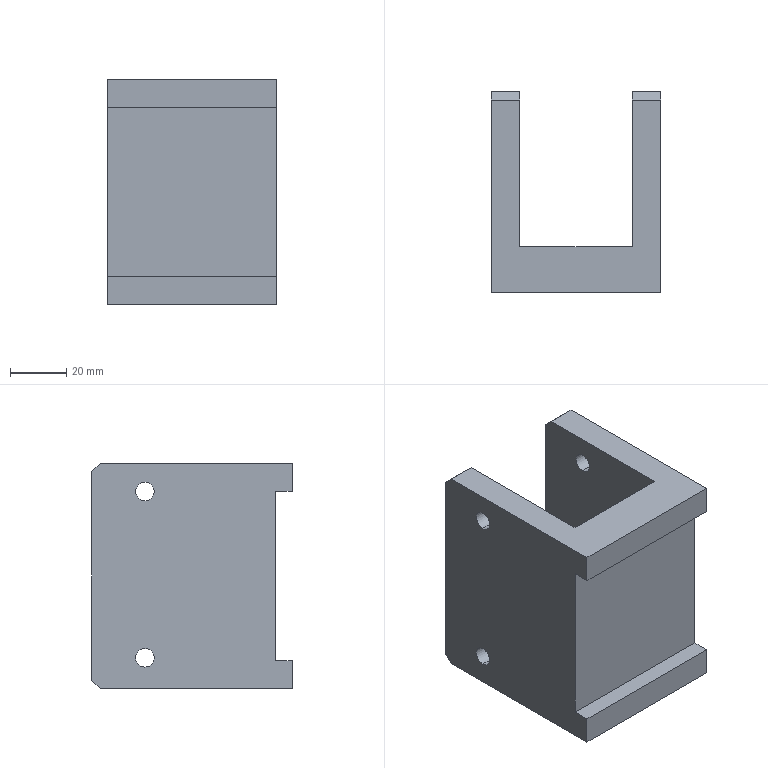Component | SolidWorks | CHEN123-AA-07-1 | 1 solid | 26 faces | box 60 x 71 x 80 mm | volume 141652 mm3 | plane 18 | cylinder 8 | commonest cylinder face diameters 6.6 x8
build123d program:
from build123d import *

# Parameters (mm, degrees)
BOSS_EXTRUDE1_DEPTH        = 80
SKETCH2_W                  = 60
SKETCH2_H                  = 6
CUT_EXTRUDE1_DEPTH         = 123.642
CHAMFER1_SIZE              = 3
F_6_6_6_6_DIAMETER_HOLE1_D = 6.6


with BuildPart() as part:
    # Sketch1 → Boss-Extrude1 (new body)
    with BuildSketch(Plane.XY):
        Polygon((-30, 0), (30, 0), (30, 71), (20, 71), (20, 16), (-20, 16), (-20, 71), (-30, 71), align=None)
    extrude(amount=BOSS_EXTRUDE1_DEPTH)

    # Sketch2 → Cut-Extrude1 (cut, through all)
    with BuildSketch(Plane.ZY.offset(30)):
        with Locations((40, 3)):
            Rectangle(SKETCH2_W, SKETCH2_H)
    extrude(amount=-CUT_EXTRUDE1_DEPTH, mode=Mode.SUBTRACT)

    # Chamfer1
    chamfer1_edges = [part.edges().sort_by_distance(p)[0] for p in [
        (25, 71, 80),
        (-25, 71, 80),
        (-25, 71, 0),
        (25, 71, 0),
    ]]
    chamfer(chamfer1_edges, length=CHAMFER1_SIZE)

    # 6.6 _6.6_ Diameter Hole1 (through all)
    with Locations(Plane(origin=(30, 0, 0), x_dir=(0, 0, -1), z_dir=(1, 0, 0))):
        with Locations((-69.874, 52.155), (-11.032, 52.155)):
            Hole(F_6_6_6_6_DIAMETER_HOLE1_D / 2)


solid = part.part

# Placed as in the assembly
solid = solid.moved(Location((-0.0005, -51.999, -137), (0, 0, 0)))
STEP:
#1=COLOUR_RGB('',0.7922,0.8196,0.9333);
#2=FILL_AREA_STYLE_COLOUR('',#1);
#3=FILL_AREA_STYLE('',(#2));
#4=SURFACE_STYLE_FILL_AREA(#3);
#5=SURFACE_SIDE_STYLE('',(#4));
#6=SURFACE_STYLE_USAGE(.BOTH.,#5);
#7=PRESENTATION_STYLE_ASSIGNMENT((#6));
#8=CARTESIAN_POINT('',(-1.181,0.006131,-2.513));
#9=VERTEX_POINT('',#8);
#10=CARTESIAN_POINT('',(-1.181,0.006131,-2.773));
#11=VERTEX_POINT('',#10);
#12=CARTESIAN_POINT('',(-1.181,0.006131,-2.643));
#13=DIRECTION('',(1.,0.,0.));
#14=DIRECTION('',(0.,0.,-1.));
#15=AXIS2_PLACEMENT_3D('',#12,#13,#14);
#16=CIRCLE('',#15,0.1299);
#17=EDGE_CURVE('',#9,#11,#16,.T.);
#18=ORIENTED_EDGE('',*,*,#17,.F.);
#19=CARTESIAN_POINT('',(-0.7874,0.006131,-2.513));
#20=VERTEX_POINT('',#19);
#21=CARTESIAN_POINT('',(1.181,0.006131,-2.513));
#22=DIRECTION('',(1.,0.,0.));
#23=VECTOR('',#22,39.37);
#24=LINE('',#21,#23);
#25=EDGE_CURVE('',#9,#20,#24,.T.);
#26=ORIENTED_EDGE('',*,*,#25,.T.);
#27=CARTESIAN_POINT('',(-0.7874,0.006131,-2.773));
#28=VERTEX_POINT('',#27);
#29=CARTESIAN_POINT('',(-0.7874,0.006131,-2.643));
#30=DIRECTION('',(-1.,0.,0.));
#31=DIRECTION('',(0.,0.,1.));
#32=AXIS2_PLACEMENT_3D('',#29,#30,#31);
#33=CIRCLE('',#32,0.1299);
#34=EDGE_CURVE('',#28,#20,#33,.T.);
#35=ORIENTED_EDGE('',*,*,#34,.F.);
#36=CARTESIAN_POINT('',(1.181,0.006131,-2.773));
#37=DIRECTION('',(1.,0.,0.));
#38=VECTOR('',#37,39.37);
#39=LINE('',#36,#38);
#40=EDGE_CURVE('',#11,#28,#39,.T.);
#41=ORIENTED_EDGE('',*,*,#40,.F.);
#42=EDGE_LOOP('',(#18,#26,#35,#41));
#43=FACE_OUTER_BOUND('',#42,.T.);
#44=CARTESIAN_POINT('',(1.181,0.006131,-2.643));
#45=DIRECTION('',(1.,0.,0.));
#46=DIRECTION('',(0.,0.,-1.));
#47=AXIS2_PLACEMENT_3D('',#44,#45,#46);
#48=CYLINDRICAL_SURFACE('',#47,0.1299);
#49=ADVANCED_FACE('',(#43),#48,.F.);
#50=CARTESIAN_POINT('',(0.7874,0.006131,-2.513));
#51=VERTEX_POINT('',#50);
#52=CARTESIAN_POINT('',(0.7874,0.006131,-2.773));
#53=VERTEX_POINT('',#52);
#54=CARTESIAN_POINT('',(0.7874,0.006131,-2.643));
#55=DIRECTION('',(1.,0.,0.));
#56=DIRECTION('',(0.,0.,-1.));
#57=AXIS2_PLACEMENT_3D('',#54,#55,#56);
#58=CIRCLE('',#57,0.1299);
#59=EDGE_CURVE('',#51,#53,#58,.T.);
#60=ORIENTED_EDGE('',*,*,#59,.F.);
#61=CARTESIAN_POINT('',(1.181,0.006131,-2.513));
#62=VERTEX_POINT('',#61);
#63=CARTESIAN_POINT('',(1.181,0.006131,-2.513));
#64=DIRECTION('',(1.,0.,0.));
#65=VECTOR('',#64,39.37);
#66=LINE('',#63,#65);
#67=EDGE_CURVE('',#51,#62,#66,.T.);
#68=ORIENTED_EDGE('',*,*,#67,.T.);
#69=CARTESIAN_POINT('',(1.181,0.006131,-2.773));
#70=VERTEX_POINT('',#69);
#71=CARTESIAN_POINT('',(1.181,0.006131,-2.643));
#72=DIRECTION('',(1.,0.,0.));
#73=DIRECTION('',(0.,0.,-1.));
#74=AXIS2_PLACEMENT_3D('',#71,#72,#73);
#75=CIRCLE('',#74,0.1299);
#76=EDGE_CURVE('',#62,#70,#75,.T.);
#77=ORIENTED_EDGE('',*,*,#76,.T.);
#78=CARTESIAN_POINT('',(1.181,0.006131,-2.773));
#79=DIRECTION('',(1.,0.,0.));
#80=VECTOR('',#79,39.37);
#81=LINE('',#78,#80);
#82=EDGE_CURVE('',#53,#70,#81,.T.);
#83=ORIENTED_EDGE('',*,*,#82,.F.);
#84=EDGE_LOOP('',(#60,#68,#77,#83));
#85=FACE_OUTER_BOUND('',#84,.T.);
#86=CARTESIAN_POINT('',(1.181,0.006131,-2.643));
#87=DIRECTION('',(1.,0.,0.));
#88=DIRECTION('',(0.,0.,-1.));
#89=AXIS2_PLACEMENT_3D('',#86,#87,#88);
#90=CYLINDRICAL_SURFACE('',#89,0.1299);
#91=ADVANCED_FACE('',(#85),#90,.F.);
#92=CARTESIAN_POINT('',(0.7874,0.006131,-4.829));
#93=VERTEX_POINT('',#92);
#94=CARTESIAN_POINT('',(0.7874,0.006131,-5.089));
#95=VERTEX_POINT('',#94);
#96=CARTESIAN_POINT('',(0.7874,0.006131,-4.959));
#97=DIRECTION('',(1.,0.,0.));
#98=DIRECTION('',(0.,0.,-1.));
#99=AXIS2_PLACEMENT_3D('',#96,#97,#98);
#100=CIRCLE('',#99,0.1299);
#101=EDGE_CURVE('',#93,#95,#100,.T.);
#102=ORIENTED_EDGE('',*,*,#101,.F.);
#103=CARTESIAN_POINT('',(1.181,0.006131,-4.829));
#104=VERTEX_POINT('',#103);
#105=CARTESIAN_POINT('',(1.181,0.006131,-4.829));
#106=DIRECTION('',(1.,0.,0.));
#107=VECTOR('',#106,39.37);
#108=LINE('',#105,#107);
#109=EDGE_CURVE('',#93,#104,#108,.T.);
#110=ORIENTED_EDGE('',*,*,#109,.T.);
#111=CARTESIAN_POINT('',(1.181,0.006131,-5.089));
#112=VERTEX_POINT('',#111);
#113=CARTESIAN_POINT('',(1.181,0.006131,-4.959));
#114=DIRECTION('',(1.,0.,0.));
#115=DIRECTION('',(0.,0.,-1.));
#116=AXIS2_PLACEMENT_3D('',#113,#114,#115);
#117=CIRCLE('',#116,0.1299);
#118=EDGE_CURVE('',#104,#112,#117,.T.);
#119=ORIENTED_EDGE('',*,*,#118,.T.);
#120=CARTESIAN_POINT('',(1.181,0.006131,-5.089));
#121=DIRECTION('',(1.,0.,0.));
#122=VECTOR('',#121,39.37);
#123=LINE('',#120,#122);
#124=EDGE_CURVE('',#95,#112,#123,.T.);
#125=ORIENTED_EDGE('',*,*,#124,.F.);
#126=EDGE_LOOP('',(#102,#110,#119,#125));
#127=FACE_OUTER_BOUND('',#126,.T.);
#128=CARTESIAN_POINT('',(1.181,0.006131,-4.959));
#129=DIRECTION('',(1.,0.,0.));
#130=DIRECTION('',(0.,0.,-1.));
#131=AXIS2_PLACEMENT_3D('',#128,#129,#130);
#132=CYLINDRICAL_SURFACE('',#131,0.1299);
#133=ADVANCED_FACE('',(#127),#132,.F.);
#134=CARTESIAN_POINT('',(-1.181,0.006131,-4.829));
#135=VERTEX_POINT('',#134);
#136=CARTESIAN_POINT('',(-1.181,0.006131,-5.089));
#137=VERTEX_POINT('',#136);
#138=CARTESIAN_POINT('',(-1.181,0.006131,-4.959));
#139=DIRECTION('',(1.,0.,0.));
#140=DIRECTION('',(0.,0.,-1.));
#141=AXIS2_PLACEMENT_3D('',#138,#139,#140);
#142=CIRCLE('',#141,0.1299);
#143=EDGE_CURVE('',#135,#137,#142,.T.);
#144=ORIENTED_EDGE('',*,*,#143,.F.);
#145=CARTESIAN_POINT('',(-0.7874,0.006131,-4.829));
#146=VERTEX_POINT('',#145);
#147=CARTESIAN_POINT('',(1.181,0.006131,-4.829));
#148=DIRECTION('',(1.,0.,0.));
#149=VECTOR('',#148,39.37);
#150=LINE('',#147,#149);
#151=EDGE_CURVE('',#135,#146,#150,.T.);
#152=ORIENTED_EDGE('',*,*,#151,.T.);
#153=CARTESIAN_POINT('',(-0.7874,0.006131,-5.089));
#154=VERTEX_POINT('',#153);
#155=CARTESIAN_POINT('',(-0.7874,0.006131,-4.959));
#156=DIRECTION('',(-1.,0.,0.));
#157=DIRECTION('',(0.,0.,1.));
#158=AXIS2_PLACEMENT_3D('',#155,#156,#157);
#159=CIRCLE('',#158,0.1299);
#160=EDGE_CURVE('',#154,#146,#159,.T.);
#161=ORIENTED_EDGE('',*,*,#160,.F.);
#162=CARTESIAN_POINT('',(1.181,0.006131,-5.089));
#163=DIRECTION('',(1.,0.,0.));
#164=VECTOR('',#163,39.37);
#165=LINE('',#162,#164);
#166=EDGE_CURVE('',#137,#154,#165,.T.);
#167=ORIENTED_EDGE('',*,*,#166,.F.);
#168=EDGE_LOOP('',(#144,#152,#161,#167));
#169=FACE_OUTER_BOUND('',#168,.T.);
#170=CARTESIAN_POINT('',(1.181,0.006131,-4.959));
#171=DIRECTION('',(1.,0.,0.));
#172=DIRECTION('',(0.,0.,-1.));
#173=AXIS2_PLACEMENT_3D('',#170,#171,#172);
#174=CYLINDRICAL_SURFACE('',#173,0.1299);
#175=ADVANCED_FACE('',(#169),#174,.F.);
#176=CARTESIAN_POINT('',(1.181,0.006131,-4.959));
#177=DIRECTION('',(1.,0.,0.));
#178=DIRECTION('',(0.,0.,-1.));
#179=AXIS2_PLACEMENT_3D('',#176,#177,#178);
#180=CIRCLE('',#179,0.1299);
#181=EDGE_CURVE('',#112,#104,#180,.T.);
#182=ORIENTED_EDGE('',*,*,#181,.F.);
#183=ORIENTED_EDGE('',*,*,#118,.F.);
#184=EDGE_LOOP('',(#182,#183));
#185=FACE_BOUND('',#184,.T.);
#186=CARTESIAN_POINT('',(1.181,-2.047,-5.394));
#187=VERTEX_POINT('',#186);
#188=CARTESIAN_POINT('',(1.181,0.63,-5.394));
#189=VERTEX_POINT('',#188);
#190=CARTESIAN_POINT('',(1.181,0.7481,-5.394));
#191=DIRECTION('',(0.,1.,0.));
#192=VECTOR('',#191,39.37);
#193=LINE('',#190,#192);
#194=EDGE_CURVE('',#187,#189,#193,.T.);
#195=ORIENTED_EDGE('',*,*,#194,.T.);
#196=CARTESIAN_POINT('',(1.181,0.7481,-5.276));
#197=VERTEX_POINT('',#196);
#198=CARTESIAN_POINT('',(1.181,0.7481,-5.276));
#199=DIRECTION('',(0.,0.7071,0.7071));
#200=VECTOR('',#199,39.37);
#201=LINE('',#198,#200);
#202=EDGE_CURVE('',#189,#197,#201,.T.);
#203=ORIENTED_EDGE('',*,*,#202,.T.);
#204=CARTESIAN_POINT('',(1.181,0.7481,-2.362));
#205=VERTEX_POINT('',#204);
#206=CARTESIAN_POINT('',(1.181,0.7481,-2.244));
#207=DIRECTION('',(0.,0.,-1.));
#208=VECTOR('',#207,39.37);
#209=LINE('',#206,#208);
#210=EDGE_CURVE('',#205,#197,#209,.T.);
#211=ORIENTED_EDGE('',*,*,#210,.F.);
#212=CARTESIAN_POINT('',(1.181,0.63,-2.244));
#213=VERTEX_POINT('',#212);
#214=CARTESIAN_POINT('',(1.181,0.63,-2.244));
#215=DIRECTION('',(-0.,-0.7071,0.7071));
#216=VECTOR('',#215,39.37);
#217=LINE('',#214,#216);
#218=EDGE_CURVE('',#205,#213,#217,.T.);
#219=ORIENTED_EDGE('',*,*,#218,.T.);
#220=CARTESIAN_POINT('',(1.181,-2.047,-2.244));
#221=VERTEX_POINT('',#220);
#222=CARTESIAN_POINT('',(1.181,0.7481,-2.244));
#223=DIRECTION('',(0.,1.,0.));
#224=VECTOR('',#223,39.37);
#225=LINE('',#222,#224);
#226=EDGE_CURVE('',#221,#213,#225,.T.);
#227=ORIENTED_EDGE('',*,*,#226,.F.);
#228=CARTESIAN_POINT('',(1.181,-2.047,-2.638));
#229=VERTEX_POINT('',#228);
#230=CARTESIAN_POINT('',(1.181,-2.047,-2.244));
#231=DIRECTION('',(0.,0.,-1.));
#232=VECTOR('',#231,39.37);
#233=LINE('',#230,#232);
#234=EDGE_CURVE('',#221,#229,#233,.T.);
#235=ORIENTED_EDGE('',*,*,#234,.T.);
#236=CARTESIAN_POINT('',(1.181,-1.811,-2.638));
#237=VERTEX_POINT('',#236);
#238=CARTESIAN_POINT('',(1.181,-2.047,-2.638));
#239=DIRECTION('',(0.,1.,0.));
#240=VECTOR('',#239,39.37);
#241=LINE('',#238,#240);
#242=EDGE_CURVE('',#229,#237,#241,.T.);
#243=ORIENTED_EDGE('',*,*,#242,.T.);
#244=CARTESIAN_POINT('',(1.181,-1.811,-5.));
#245=VERTEX_POINT('',#244);
#246=CARTESIAN_POINT('',(1.181,-1.811,-5.));
#247=DIRECTION('',(0.,0.,-1.));
#248=VECTOR('',#247,39.37);
#249=LINE('',#246,#248);
#250=EDGE_CURVE('',#237,#245,#249,.T.);
#251=ORIENTED_EDGE('',*,*,#250,.T.);
#252=CARTESIAN_POINT('',(1.181,-2.047,-5.));
#253=VERTEX_POINT('',#252);
#254=CARTESIAN_POINT('',(1.181,-2.047,-5.));
#255=DIRECTION('',(0.,-1.,-0.));
#256=VECTOR('',#255,39.37);
#257=LINE('',#254,#256);
#258=EDGE_CURVE('',#245,#253,#257,.T.);
#259=ORIENTED_EDGE('',*,*,#258,.T.);
#260=CARTESIAN_POINT('',(1.181,-2.047,-2.244));
#261=DIRECTION('',(0.,0.,-1.));
#262=VECTOR('',#261,39.37);
#263=LINE('',#260,#262);
#264=EDGE_CURVE('',#253,#187,#263,.T.);
#265=ORIENTED_EDGE('',*,*,#264,.T.);
#266=EDGE_LOOP('',(#195,#203,#211,#219,#227,#235,#243,#251,#259,#265));
#267=FACE_OUTER_BOUND('',#266,.T.);
#268=CARTESIAN_POINT('',(1.181,0.006131,-2.643));
#269=DIRECTION('',(1.,0.,0.));
#270=DIRECTION('',(0.,0.,-1.));
#271=AXIS2_PLACEMENT_3D('',#268,#269,#270);
#272=CIRCLE('',#271,0.1299);
#273=EDGE_CURVE('',#70,#62,#272,.T.);
#274=ORIENTED_EDGE('',*,*,#273,.F.);
#275=ORIENTED_EDGE('',*,*,#76,.F.);
#276=EDGE_LOOP('',(#274,#275));
#277=FACE_BOUND('',#276,.T.);
#278=CARTESIAN_POINT('',(1.181,0.7481,-2.244));
#279=DIRECTION('',(-1.,0.,0.));
#280=DIRECTION('',(-0.,-1.,0.));
#281=AXIS2_PLACEMENT_3D('',#278,#279,#280);
#282=PLANE('',#281);
#283=ADVANCED_FACE('',(#185,#267,#277),#282,.F.);
#284=ORIENTED_EDGE('',*,*,#264,.F.);
#285=CARTESIAN_POINT('',(-1.181,-2.047,-5.));
#286=VERTEX_POINT('',#285);
#287=CARTESIAN_POINT('',(1.181,-2.047,-5.));
#288=DIRECTION('',(-1.,0.,0.));
#289=VECTOR('',#288,39.37);
#290=LINE('',#287,#289);
#291=EDGE_CURVE('',#253,#286,#290,.T.);
#292=ORIENTED_EDGE('',*,*,#291,.T.);
#293=CARTESIAN_POINT('',(-1.181,-2.047,-5.394));
#294=VERTEX_POINT('',#293);
#295=CARTESIAN_POINT('',(-1.181,-2.047,-2.244));
#296=DIRECTION('',(0.,0.,-1.));
#297=VECTOR('',#296,39.37);
#298=LINE('',#295,#297);
#299=EDGE_CURVE('',#286,#294,#298,.T.);
#300=ORIENTED_EDGE('',*,*,#299,.T.);
#301=CARTESIAN_POINT('',(-1.181,-2.047,-5.394));
#302=DIRECTION('',(1.,0.,0.));
#303=VECTOR('',#302,39.37);
#304=LINE('',#301,#303);
#305=EDGE_CURVE('',#294,#187,#304,.T.);
#306=ORIENTED_EDGE('',*,*,#305,.T.);
#307=EDGE_LOOP('',(#284,#292,#300,#306));
#308=FACE_OUTER_BOUND('',#307,.T.);
#309=CARTESIAN_POINT('',(-1.181,-2.047,-2.244));
#310=DIRECTION('',(0.,1.,0.));
#311=DIRECTION('',(0.,0.,1.));
#312=AXIS2_PLACEMENT_3D('',#309,#310,#311);
#313=PLANE('',#312);
#314=ADVANCED_FACE('',(#308),#313,.F.);
#315=CARTESIAN_POINT('',(-1.181,0.006131,-2.643));
#316=DIRECTION('',(1.,0.,0.));
#317=DIRECTION('',(0.,0.,-1.));
#318=AXIS2_PLACEMENT_3D('',#315,#316,#317);
#319=CIRCLE('',#318,0.1299);
#320=EDGE_CURVE('',#11,#9,#319,.T.);
#321=ORIENTED_EDGE('',*,*,#320,.T.);
#322=ORIENTED_EDGE('',*,*,#17,.T.);
#323=EDGE_LOOP('',(#321,#322));
#324=FACE_BOUND('',#323,.T.);
#325=CARTESIAN_POINT('',(-1.181,0.006131,-4.959));
#326=DIRECTION('',(1.,0.,0.));
#327=DIRECTION('',(0.,0.,-1.));
#328=AXIS2_PLACEMENT_3D('',#325,#326,#327);
#329=CIRCLE('',#328,0.1299);
#330=EDGE_CURVE('',#137,#135,#329,.T.);
#331=ORIENTED_EDGE('',*,*,#330,.T.);
#332=ORIENTED_EDGE('',*,*,#143,.T.);
#333=EDGE_LOOP('',(#331,#332));
#334=FACE_BOUND('',#333,.T.);
#335=CARTESIAN_POINT('',(-1.181,0.7481,-2.362));
#336=VERTEX_POINT('',#335);
#337=CARTESIAN_POINT('',(-1.181,0.7481,-5.276));
#338=VERTEX_POINT('',#337);
#339=CARTESIAN_POINT('',(-1.181,0.7481,-2.244));
#340=DIRECTION('',(0.,0.,-1.));
#341=VECTOR('',#340,39.37);
#342=LINE('',#339,#341);
#343=EDGE_CURVE('',#336,#338,#342,.T.);
#344=ORIENTED_EDGE('',*,*,#343,.T.);
#345=CARTESIAN_POINT('',(-1.181,0.63,-5.394));
#346=VERTEX_POINT('',#345);
#347=CARTESIAN_POINT('',(-1.181,0.7481,-5.276));
#348=DIRECTION('',(0.,-0.7071,-0.7071));
#349=VECTOR('',#348,39.37);
#350=LINE('',#347,#349);
#351=EDGE_CURVE('',#338,#346,#350,.T.);
#352=ORIENTED_EDGE('',*,*,#351,.T.);
#353=CARTESIAN_POINT('',(-1.181,-2.047,-5.394));
#354=DIRECTION('',(0.,-1.,0.));
#355=VECTOR('',#354,39.37);
#356=LINE('',#353,#355);
#357=EDGE_CURVE('',#346,#294,#356,.T.);
#358=ORIENTED_EDGE('',*,*,#357,.T.);
#359=ORIENTED_EDGE('',*,*,#299,.F.);
#360=CARTESIAN_POINT('',(-1.181,-1.811,-5.));
#361=VERTEX_POINT('',#360);
#362=CARTESIAN_POINT('',(-1.181,-2.047,-5.));
#363=DIRECTION('',(0.,-1.,-0.));
#364=VECTOR('',#363,39.37);
#365=LINE('',#362,#364);
#366=EDGE_CURVE('',#361,#286,#365,.T.);
#367=ORIENTED_EDGE('',*,*,#366,.F.);
#368=CARTESIAN_POINT('',(-1.181,-1.811,-2.638));
#369=VERTEX_POINT('',#368);
#370=CARTESIAN_POINT('',(-1.181,-1.811,-5.));
#371=DIRECTION('',(0.,0.,-1.));
#372=VECTOR('',#371,39.37);
#373=LINE('',#370,#372);
#374=EDGE_CURVE('',#369,#361,#373,.T.);
#375=ORIENTED_EDGE('',*,*,#374,.F.);
#376=CARTESIAN_POINT('',(-1.181,-2.047,-2.638));
#377=VERTEX_POINT('',#376);
#378=CARTESIAN_POINT('',(-1.181,-2.047,-2.638));
#379=DIRECTION('',(0.,1.,0.));
#380=VECTOR('',#379,39.37);
#381=LINE('',#378,#380);
#382=EDGE_CURVE('',#377,#369,#381,.T.);
#383=ORIENTED_EDGE('',*,*,#382,.F.);
#384=CARTESIAN_POINT('',(-1.181,-2.047,-2.244));
#385=VERTEX_POINT('',#384);
#386=CARTESIAN_POINT('',(-1.181,-2.047,-2.244));
#387=DIRECTION('',(0.,0.,-1.));
#388=VECTOR('',#387,39.37);
#389=LINE('',#386,#388);
#390=EDGE_CURVE('',#385,#377,#389,.T.);
#391=ORIENTED_EDGE('',*,*,#390,.F.);
#392=CARTESIAN_POINT('',(-1.181,0.63,-2.244));
#393=VERTEX_POINT('',#392);
#394=CARTESIAN_POINT('',(-1.181,-2.047,-2.244));
#395=DIRECTION('',(0.,-1.,0.));
#396=VECTOR('',#395,39.37);
#397=LINE('',#394,#396);
#398=EDGE_CURVE('',#393,#385,#397,.T.);
#399=ORIENTED_EDGE('',*,*,#398,.F.);
#400=CARTESIAN_POINT('',(-1.181,0.63,-2.244));
#401=DIRECTION('',(0.,0.7071,-0.7071));
#402=VECTOR('',#401,39.37);
#403=LINE('',#400,#402);
#404=EDGE_CURVE('',#393,#336,#403,.T.);
#405=ORIENTED_EDGE('',*,*,#404,.T.);
#406=EDGE_LOOP('',(#344,#352,#358,#359,#367,#375,#383,#391,#399,#405));
#407=FACE_OUTER_BOUND('',#406,.T.);
#408=CARTESIAN_POINT('',(-1.181,-2.047,-2.244));
#409=DIRECTION('',(1.,0.,0.));
#410=DIRECTION('',(0.,0.,-1.));
#411=AXIS2_PLACEMENT_3D('',#408,#409,#410);
#412=PLANE('',#411);
#413=ADVANCED_FACE('',(#324,#334,#407),#412,.F.);
#414=ORIENTED_EDGE('',*,*,#390,.T.);
#415=CARTESIAN_POINT('',(1.181,-2.047,-2.638));
#416=DIRECTION('',(-1.,0.,0.));
#417=VECTOR('',#416,39.37);
#418=LINE('',#415,#417);
#419=EDGE_CURVE('',#229,#377,#418,.T.);
#420=ORIENTED_EDGE('',*,*,#419,.F.);
#421=ORIENTED_EDGE('',*,*,#234,.F.);
#422=CARTESIAN_POINT('',(-1.181,-2.047,-2.244));
#423=DIRECTION('',(1.,0.,0.));
#424=VECTOR('',#423,39.37);
#425=LINE('',#422,#424);
#426=EDGE_CURVE('',#385,#221,#425,.T.);
#427=ORIENTED_EDGE('',*,*,#426,.F.);
#428=EDGE_LOOP('',(#414,#420,#421,#427));
#429=FACE_OUTER_BOUND('',#428,.T.);
#430=CARTESIAN_POINT('',(-1.181,-2.047,-2.244));
#431=DIRECTION('',(0.,1.,0.));
#432=DIRECTION('',(0.,0.,1.));
#433=AXIS2_PLACEMENT_3D('',#430,#431,#432);
#434=PLANE('',#433);
#435=ADVANCED_FACE('',(#429),#434,.F.);
#436=ORIENTED_EDGE('',*,*,#210,.T.);
#437=CARTESIAN_POINT('',(0.7874,0.7481,-5.276));
#438=VERTEX_POINT('',#437);
#439=CARTESIAN_POINT('',(0.7874,0.7481,-5.276));
#440=DIRECTION('',(-1.,0.,0.));
#441=VECTOR('',#440,39.37);
#442=LINE('',#439,#441);
#443=EDGE_CURVE('',#197,#438,#442,.T.);
#444=ORIENTED_EDGE('',*,*,#443,.T.);
#445=CARTESIAN_POINT('',(0.7874,0.7481,-2.362));
#446=VERTEX_POINT('',#445);
#447=CARTESIAN_POINT('',(0.7874,0.7481,-2.244));
#448=DIRECTION('',(0.,0.,-1.));
#449=VECTOR('',#448,39.37);
#450=LINE('',#447,#449);
#451=EDGE_CURVE('',#446,#438,#450,.T.);
#452=ORIENTED_EDGE('',*,*,#451,.F.);
#453=CARTESIAN_POINT('',(0.7874,0.7481,-2.362));
#454=DIRECTION('',(1.,0.,0.));
#455=VECTOR('',#454,39.37);
#456=LINE('',#453,#455);
#457=EDGE_CURVE('',#446,#205,#456,.T.);
#458=ORIENTED_EDGE('',*,*,#457,.T.);
#459=EDGE_LOOP('',(#436,#444,#452,#458));
#460=FACE_OUTER_BOUND('',#459,.T.);
#461=CARTESIAN_POINT('',(0.7874,0.7481,-2.244));
#462=DIRECTION('',(0.,-1.,0.));
#463=DIRECTION('',(0.,0.,-1.));
#464=AXIS2_PLACEMENT_3D('',#461,#462,#463);
#465=PLANE('',#464);
#466=ADVANCED_FACE('',(#460),#465,.F.);
#467=CARTESIAN_POINT('',(0.7874,0.006131,-2.643));
#468=DIRECTION('',(1.,0.,0.));
#469=DIRECTION('',(0.,0.,-1.));
#470=AXIS2_PLACEMENT_3D('',#467,#468,#469);
#471=CIRCLE('',#470,0.1299);
#472=EDGE_CURVE('',#53,#51,#471,.T.);
#473=ORIENTED_EDGE('',*,*,#472,.T.);
#474=ORIENTED_EDGE('',*,*,#59,.T.);
#475=EDGE_LOOP('',(#473,#474));
#476=FACE_BOUND('',#475,.T.);
#477=CARTESIAN_POINT('',(0.7874,0.006131,-4.959));
#478=DIRECTION('',(1.,0.,0.));
#479=DIRECTION('',(0.,0.,-1.));
#480=AXIS2_PLACEMENT_3D('',#477,#478,#479);
#481=CIRCLE('',#480,0.1299);
#482=EDGE_CURVE('',#95,#93,#481,.T.);
#483=ORIENTED_EDGE('',*,*,#482,.T.);
#484=ORIENTED_EDGE('',*,*,#101,.T.);
#485=EDGE_LOOP('',(#483,#484));
#486=FACE_BOUND('',#485,.T.);
#487=ORIENTED_EDGE('',*,*,#451,.T.);
#488=CARTESIAN_POINT('',(0.7874,0.63,-5.394));
#489=VERTEX_POINT('',#488);
#490=CARTESIAN_POINT('',(0.7874,0.7481,-5.276));
#491=DIRECTION('',(0.,-0.7071,-0.7071));
#492=VECTOR('',#491,39.37);
#493=LINE('',#490,#492);
#494=EDGE_CURVE('',#438,#489,#493,.T.);
#495=ORIENTED_EDGE('',*,*,#494,.T.);
#496=CARTESIAN_POINT('',(0.7874,-1.417,-5.394));
#497=VERTEX_POINT('',#496);
#498=CARTESIAN_POINT('',(0.7874,-1.417,-5.394));
#499=DIRECTION('',(0.,-1.,0.));
#500=VECTOR('',#499,39.37);
#501=LINE('',#498,#500);
#502=EDGE_CURVE('',#489,#497,#501,.T.);
#503=ORIENTED_EDGE('',*,*,#502,.T.);
#504=CARTESIAN_POINT('',(0.7874,-1.417,-2.244));
#505=VERTEX_POINT('',#504);
#506=CARTESIAN_POINT('',(0.7874,-1.417,-2.244));
#507=DIRECTION('',(0.,0.,-1.));
#508=VECTOR('',#507,39.37);
#509=LINE('',#506,#508);
#510=EDGE_CURVE('',#505,#497,#509,.T.);
#511=ORIENTED_EDGE('',*,*,#510,.F.);
#512=CARTESIAN_POINT('',(0.7874,0.63,-2.244));
#513=VERTEX_POINT('',#512);
#514=CARTESIAN_POINT('',(0.7874,-1.417,-2.244));
#515=DIRECTION('',(0.,-1.,0.));
#516=VECTOR('',#515,39.37);
#517=LINE('',#514,#516);
#518=EDGE_CURVE('',#513,#505,#517,.T.);
#519=ORIENTED_EDGE('',*,*,#518,.F.);
#520=CARTESIAN_POINT('',(0.7874,0.63,-2.244));
#521=DIRECTION('',(0.,0.7071,-0.7071));
#522=VECTOR('',#521,39.37);
#523=LINE('',#520,#522);
#524=EDGE_CURVE('',#513,#446,#523,.T.);
#525=ORIENTED_EDGE('',*,*,#524,.T.);
#526=EDGE_LOOP('',(#487,#495,#503,#511,#519,#525));
#527=FACE_OUTER_BOUND('',#526,.T.);
#528=CARTESIAN_POINT('',(0.7874,-1.417,-2.244));
#529=DIRECTION('',(1.,0.,0.));
#530=DIRECTION('',(0.,0.,-1.));
#531=AXIS2_PLACEMENT_3D('',#528,#529,#530);
#532=PLANE('',#531);
#533=ADVANCED_FACE('',(#476,#486,#527),#532,.F.);
#534=CARTESIAN_POINT('',(-0.7874,-1.417,-5.394));
#535=VERTEX_POINT('',#534);
#536=CARTESIAN_POINT('',(-0.7874,-1.417,-5.394));
#537=DIRECTION('',(-1.,-0.,0.));
#538=VECTOR('',#537,39.37);
#539=LINE('',#536,#538);
#540=EDGE_CURVE('',#497,#535,#539,.T.);
#541=ORIENTED_EDGE('',*,*,#540,.T.);
#542=CARTESIAN_POINT('',(-0.7874,-1.417,-2.244));
#543=VERTEX_POINT('',#542);
#544=CARTESIAN_POINT('',(-0.7874,-1.417,-2.244));
#545=DIRECTION('',(0.,0.,-1.));
#546=VECTOR('',#545,39.37);
#547=LINE('',#544,#546);
#548=EDGE_CURVE('',#543,#535,#547,.T.);
#549=ORIENTED_EDGE('',*,*,#548,.F.);
#550=CARTESIAN_POINT('',(-0.7874,-1.417,-2.244));
#551=DIRECTION('',(-1.,-0.,0.));
#552=VECTOR('',#551,39.37);
#553=LINE('',#550,#552);
#554=EDGE_CURVE('',#505,#543,#553,.T.);
#555=ORIENTED_EDGE('',*,*,#554,.F.);
#556=ORIENTED_EDGE('',*,*,#510,.T.);
#557=EDGE_LOOP('',(#541,#549,#555,#556));
#558=FACE_OUTER_BOUND('',#557,.T.);
#559=CARTESIAN_POINT('',(-0.7874,-1.417,-2.244));
#560=DIRECTION('',(0.,-1.,0.));
#561=DIRECTION('',(1.,0.,0.));
#562=AXIS2_PLACEMENT_3D('',#559,#560,#561);
#563=PLANE('',#562);
#564=ADVANCED_FACE('',(#558),#563,.F.);
#565=ORIENTED_EDGE('',*,*,#34,.T.);
#566=CARTESIAN_POINT('',(-0.7874,0.006131,-2.643));
#567=DIRECTION('',(-1.,0.,0.));
#568=DIRECTION('',(0.,0.,1.));
#569=AXIS2_PLACEMENT_3D('',#566,#567,#568);
#570=CIRCLE('',#569,0.1299);
#571=EDGE_CURVE('',#20,#28,#570,.T.);
#572=ORIENTED_EDGE('',*,*,#571,.T.);
#573=EDGE_LOOP('',(#565,#572));
#574=FACE_BOUND('',#573,.T.);
#575=ORIENTED_EDGE('',*,*,#160,.T.);
#576=CARTESIAN_POINT('',(-0.7874,0.006131,-4.959));
#577=DIRECTION('',(-1.,0.,0.));
#578=DIRECTION('',(0.,0.,1.));
#579=AXIS2_PLACEMENT_3D('',#576,#577,#578);
#580=CIRCLE('',#579,0.1299);
#581=EDGE_CURVE('',#146,#154,#580,.T.);
#582=ORIENTED_EDGE('',*,*,#581,.T.);
#583=EDGE_LOOP('',(#575,#582));
#584=FACE_BOUND('',#583,.T.);
#585=CARTESIAN_POINT('',(-0.7874,0.63,-5.394));
#586=VERTEX_POINT('',#585);
#587=CARTESIAN_POINT('',(-0.7874,0.7481,-5.394));
#588=DIRECTION('',(0.,1.,0.));
#589=VECTOR('',#588,39.37);
#590=LINE('',#587,#589);
#591=EDGE_CURVE('',#535,#586,#590,.T.);
#592=ORIENTED_EDGE('',*,*,#591,.T.);
#593=CARTESIAN_POINT('',(-0.7874,0.7481,-5.276));
#594=VERTEX_POINT('',#593);
#595=CARTESIAN_POINT('',(-0.7874,0.7481,-5.276));
#596=DIRECTION('',(0.,0.7071,0.7071));
#597=VECTOR('',#596,39.37);
#598=LINE('',#595,#597);
#599=EDGE_CURVE('',#586,#594,#598,.T.);
#600=ORIENTED_EDGE('',*,*,#599,.T.);
#601=CARTESIAN_POINT('',(-0.7874,0.7481,-2.362));
#602=VERTEX_POINT('',#601);
#603=CARTESIAN_POINT('',(-0.7874,0.7481,-2.244));
#604=DIRECTION('',(0.,0.,-1.));
#605=VECTOR('',#604,39.37);
#606=LINE('',#603,#605);
#607=EDGE_CURVE('',#602,#594,#606,.T.);
#608=ORIENTED_EDGE('',*,*,#607,.F.);
#609=CARTESIAN_POINT('',(-0.7874,0.63,-2.244));
#610=VERTEX_POINT('',#609);
#611=CARTESIAN_POINT('',(-0.7874,0.63,-2.244));
#612=DIRECTION('',(0.,-0.7071,0.7071));
#613=VECTOR('',#612,39.37);
#614=LINE('',#611,#613);
#615=EDGE_CURVE('',#602,#610,#614,.T.);
#616=ORIENTED_EDGE('',*,*,#615,.T.);
#617=CARTESIAN_POINT('',(-0.7874,0.7481,-2.244));
#618=DIRECTION('',(0.,1.,0.));
#619=VECTOR('',#618,39.37);
#620=LINE('',#617,#619);
#621=EDGE_CURVE('',#543,#610,#620,.T.);
#622=ORIENTED_EDGE('',*,*,#621,.F.);
#623=ORIENTED_EDGE('',*,*,#548,.T.);
#624=EDGE_LOOP('',(#592,#600,#608,#616,#622,#623));
#625=FACE_OUTER_BOUND('',#624,.T.);
#626=CARTESIAN_POINT('',(-0.7874,0.7481,-2.244));
#627=DIRECTION('',(-1.,0.,0.));
#628=DIRECTION('',(0.,0.,1.));
#629=AXIS2_PLACEMENT_3D('',#626,#627,#628);
#630=PLANE('',#629);
#631=ADVANCED_FACE('',(#574,#584,#625),#630,.F.);
#632=ORIENTED_EDGE('',*,*,#607,.T.);
#633=CARTESIAN_POINT('',(-1.181,0.7481,-5.276));
#634=DIRECTION('',(-1.,0.,0.));
#635=VECTOR('',#634,39.37);
#636=LINE('',#633,#635);
#637=EDGE_CURVE('',#594,#338,#636,.T.);
#638=ORIENTED_EDGE('',*,*,#637,.T.);
#639=ORIENTED_EDGE('',*,*,#343,.F.);
#640=CARTESIAN_POINT('',(-1.181,0.7481,-2.362));
#641=DIRECTION('',(1.,0.,0.));
#642=VECTOR('',#641,39.37);
#643=LINE('',#640,#642);
#644=EDGE_CURVE('',#336,#602,#643,.T.);
#645=ORIENTED_EDGE('',*,*,#644,.T.);
#646=EDGE_LOOP('',(#632,#638,#639,#645));
#647=FACE_OUTER_BOUND('',#646,.T.);
#648=CARTESIAN_POINT('',(-1.181,0.7481,-2.244));
#649=DIRECTION('',(0.,-1.,0.));
#650=DIRECTION('',(0.,0.,-1.));
#651=AXIS2_PLACEMENT_3D('',#648,#649,#650);
#652=PLANE('',#651);
#653=ADVANCED_FACE('',(#647),#652,.F.);
#654=ORIENTED_EDGE('',*,*,#621,.T.);
#655=CARTESIAN_POINT('',(-0.00001969,0.63,-2.244));
#656=DIRECTION('',(-1.,0.,0.));
#657=VECTOR('',#656,39.37);
#658=LINE('',#655,#657);
#659=EDGE_CURVE('',#610,#393,#658,.T.);
#660=ORIENTED_EDGE('',*,*,#659,.T.);
#661=ORIENTED_EDGE('',*,*,#398,.T.);
#662=ORIENTED_EDGE('',*,*,#426,.T.);
#663=ORIENTED_EDGE('',*,*,#226,.T.);
#664=CARTESIAN_POINT('',(-0.00001969,0.63,-2.244));
#665=DIRECTION('',(-1.,0.,0.));
#666=VECTOR('',#665,39.37);
#667=LINE('',#664,#666);
#668=EDGE_CURVE('',#213,#513,#667,.T.);
#669=ORIENTED_EDGE('',*,*,#668,.T.);
#670=ORIENTED_EDGE('',*,*,#518,.T.);
#671=ORIENTED_EDGE('',*,*,#554,.T.);
#672=EDGE_LOOP('',(#654,#660,#661,#662,#663,#669,#670,#671));
#673=FACE_OUTER_BOUND('',#672,.T.);
#674=CARTESIAN_POINT('',(-0.00001969,-2.047,-2.244));
#675=DIRECTION('',(0.,0.,-1.));
#676=DIRECTION('',(-1.,0.,0.));
#677=AXIS2_PLACEMENT_3D('',#674,#675,#676);
#678=PLANE('',#677);
#679=ADVANCED_FACE('',(#673),#678,.F.);
#680=ORIENTED_EDGE('',*,*,#502,.F.);
#681=CARTESIAN_POINT('',(1.181,0.63,-5.394));
#682=DIRECTION('',(1.,0.,0.));
#683=VECTOR('',#682,39.37);
#684=LINE('',#681,#683);
#685=EDGE_CURVE('',#489,#189,#684,.T.);
#686=ORIENTED_EDGE('',*,*,#685,.T.);
#687=ORIENTED_EDGE('',*,*,#194,.F.);
#688=ORIENTED_EDGE('',*,*,#305,.F.);
#689=ORIENTED_EDGE('',*,*,#357,.F.);
#690=CARTESIAN_POINT('',(-0.7874,0.63,-5.394));
#691=DIRECTION('',(1.,0.,0.));
#692=VECTOR('',#691,39.37);
#693=LINE('',#690,#692);
#694=EDGE_CURVE('',#346,#586,#693,.T.);
#695=ORIENTED_EDGE('',*,*,#694,.T.);
#696=ORIENTED_EDGE('',*,*,#591,.F.);
#697=ORIENTED_EDGE('',*,*,#540,.F.);
#698=EDGE_LOOP('',(#680,#686,#687,#688,#689,#695,#696,#697));
#699=FACE_OUTER_BOUND('',#698,.T.);
#700=CARTESIAN_POINT('',(-0.00001969,-2.047,-5.394));
#701=DIRECTION('',(0.,0.,-1.));
#702=DIRECTION('',(-1.,0.,0.));
#703=AXIS2_PLACEMENT_3D('',#700,#701,#702);
#704=PLANE('',#703);
#705=ADVANCED_FACE('',(#699),#704,.T.);
#706=ORIENTED_EDGE('',*,*,#366,.T.);
#707=ORIENTED_EDGE('',*,*,#291,.F.);
#708=ORIENTED_EDGE('',*,*,#258,.F.);
#709=CARTESIAN_POINT('',(1.181,-1.811,-5.));
#710=DIRECTION('',(-1.,0.,0.));
#711=VECTOR('',#710,39.37);
#712=LINE('',#709,#711);
#713=EDGE_CURVE('',#245,#361,#712,.T.);
#714=ORIENTED_EDGE('',*,*,#713,.T.);
#715=EDGE_LOOP('',(#706,#707,#708,#714));
#716=FACE_OUTER_BOUND('',#715,.T.);
#717=CARTESIAN_POINT('',(1.181,-2.047,-5.));
#718=DIRECTION('',(0.,0.,-1.));
#719=DIRECTION('',(0.,1.,0.));
#720=AXIS2_PLACEMENT_3D('',#717,#718,#719);
#721=PLANE('',#720);
#722=ADVANCED_FACE('',(#716),#721,.F.);
#723=ORIENTED_EDGE('',*,*,#374,.T.);
#724=ORIENTED_EDGE('',*,*,#713,.F.);
#725=ORIENTED_EDGE('',*,*,#250,.F.);
#726=CARTESIAN_POINT('',(1.181,-1.811,-2.638));
#727=DIRECTION('',(-1.,0.,0.));
#728=VECTOR('',#727,39.37);
#729=LINE('',#726,#728);
#730=EDGE_CURVE('',#237,#369,#729,.T.);
#731=ORIENTED_EDGE('',*,*,#730,.T.);
#732=EDGE_LOOP('',(#723,#724,#725,#731));
#733=FACE_OUTER_BOUND('',#732,.T.);
#734=CARTESIAN_POINT('',(1.181,-1.811,-5.));
#735=DIRECTION('',(0.,1.,0.));
#736=DIRECTION('',(0.,0.,1.));
#737=AXIS2_PLACEMENT_3D('',#734,#735,#736);
#738=PLANE('',#737);
#739=ADVANCED_FACE('',(#733),#738,.F.);
#740=ORIENTED_EDGE('',*,*,#382,.T.);
#741=ORIENTED_EDGE('',*,*,#730,.F.);
#742=ORIENTED_EDGE('',*,*,#242,.F.);
#743=ORIENTED_EDGE('',*,*,#419,.T.);
#744=EDGE_LOOP('',(#740,#741,#742,#743));
#745=FACE_OUTER_BOUND('',#744,.T.);
#746=CARTESIAN_POINT('',(1.181,-2.047,-2.638));
#747=DIRECTION('',(0.,0.,1.));
#748=DIRECTION('',(1.,0.,0.));
#749=AXIS2_PLACEMENT_3D('',#746,#747,#748);
#750=PLANE('',#749);
#751=ADVANCED_FACE('',(#745),#750,.F.);
#752=ORIENTED_EDGE('',*,*,#202,.F.);
#753=ORIENTED_EDGE('',*,*,#685,.F.);
#754=ORIENTED_EDGE('',*,*,#494,.F.);
#755=ORIENTED_EDGE('',*,*,#443,.F.);
#756=EDGE_LOOP('',(#752,#753,#754,#755));
#757=FACE_OUTER_BOUND('',#756,.T.);
#758=CARTESIAN_POINT('',(0.7874,0.7481,-5.276));
#759=DIRECTION('',(0.,0.7071,-0.7071));
#760=DIRECTION('',(1.,0.,0.));
#761=AXIS2_PLACEMENT_3D('',#758,#759,#760);
#762=PLANE('',#761);
#763=ADVANCED_FACE('',(#757),#762,.T.);
#764=ORIENTED_EDGE('',*,*,#599,.F.);
#765=ORIENTED_EDGE('',*,*,#694,.F.);
#766=ORIENTED_EDGE('',*,*,#351,.F.);
#767=ORIENTED_EDGE('',*,*,#637,.F.);
#768=EDGE_LOOP('',(#764,#765,#766,#767));
#769=FACE_OUTER_BOUND('',#768,.T.);
#770=CARTESIAN_POINT('',(-1.181,0.7481,-5.276));
#771=DIRECTION('',(0.,0.7071,-0.7071));
#772=DIRECTION('',(1.,0.,0.));
#773=AXIS2_PLACEMENT_3D('',#770,#771,#772);
#774=PLANE('',#773);
#775=ADVANCED_FACE('',(#769),#774,.T.);
#776=ORIENTED_EDGE('',*,*,#615,.F.);
#777=ORIENTED_EDGE('',*,*,#644,.F.);
#778=ORIENTED_EDGE('',*,*,#404,.F.);
#779=ORIENTED_EDGE('',*,*,#659,.F.);
#780=EDGE_LOOP('',(#776,#777,#778,#779));
#781=FACE_OUTER_BOUND('',#780,.T.);
#782=CARTESIAN_POINT('',(-0.00001969,0.63,-2.244));
#783=DIRECTION('',(0.,-0.7071,-0.7071));
#784=DIRECTION('',(-1.,0.,0.));
#785=AXIS2_PLACEMENT_3D('',#782,#783,#784);
#786=PLANE('',#785);
#787=ADVANCED_FACE('',(#781),#786,.F.);
#788=ORIENTED_EDGE('',*,*,#218,.F.);
#789=ORIENTED_EDGE('',*,*,#457,.F.);
#790=ORIENTED_EDGE('',*,*,#524,.F.);
#791=ORIENTED_EDGE('',*,*,#668,.F.);
#792=EDGE_LOOP('',(#788,#789,#790,#791));
#793=FACE_OUTER_BOUND('',#792,.T.);
#794=CARTESIAN_POINT('',(-0.00001969,0.63,-2.244));
#795=DIRECTION('',(0.,-0.7071,-0.7071));
#796=DIRECTION('',(-1.,0.,0.));
#797=AXIS2_PLACEMENT_3D('',#794,#795,#796);
#798=PLANE('',#797);
#799=ADVANCED_FACE('',(#793),#798,.F.);
#800=ORIENTED_EDGE('',*,*,#151,.F.);
#801=ORIENTED_EDGE('',*,*,#330,.F.);
#802=ORIENTED_EDGE('',*,*,#166,.T.);
#803=ORIENTED_EDGE('',*,*,#581,.F.);
#804=EDGE_LOOP('',(#800,#801,#802,#803));
#805=FACE_OUTER_BOUND('',#804,.T.);
#806=CARTESIAN_POINT('',(1.181,0.006131,-4.959));
#807=DIRECTION('',(1.,0.,0.));
#808=DIRECTION('',(0.,0.,-1.));
#809=AXIS2_PLACEMENT_3D('',#806,#807,#808);
#810=CYLINDRICAL_SURFACE('',#809,0.1299);
#811=ADVANCED_FACE('',(#805),#810,.F.);
#812=ORIENTED_EDGE('',*,*,#109,.F.);
#813=ORIENTED_EDGE('',*,*,#482,.F.);
#814=ORIENTED_EDGE('',*,*,#124,.T.);
#815=ORIENTED_EDGE('',*,*,#181,.T.);
#816=EDGE_LOOP('',(#812,#813,#814,#815));
#817=FACE_OUTER_BOUND('',#816,.T.);
#818=CARTESIAN_POINT('',(1.181,0.006131,-4.959));
#819=DIRECTION('',(1.,0.,0.));
#820=DIRECTION('',(0.,0.,-1.));
#821=AXIS2_PLACEMENT_3D('',#818,#819,#820);
#822=CYLINDRICAL_SURFACE('',#821,0.1299);
#823=ADVANCED_FACE('',(#817),#822,.F.);
#824=ORIENTED_EDGE('',*,*,#67,.F.);
#825=ORIENTED_EDGE('',*,*,#472,.F.);
#826=ORIENTED_EDGE('',*,*,#82,.T.);
#827=ORIENTED_EDGE('',*,*,#273,.T.);
#828=EDGE_LOOP('',(#824,#825,#826,#827));
#829=FACE_OUTER_BOUND('',#828,.T.);
#830=CARTESIAN_POINT('',(1.181,0.006131,-2.643));
#831=DIRECTION('',(1.,0.,0.));
#832=DIRECTION('',(0.,0.,-1.));
#833=AXIS2_PLACEMENT_3D('',#830,#831,#832);
#834=CYLINDRICAL_SURFACE('',#833,0.1299);
#835=ADVANCED_FACE('',(#829),#834,.F.);
#836=ORIENTED_EDGE('',*,*,#25,.F.);
#837=ORIENTED_EDGE('',*,*,#320,.F.);
#838=ORIENTED_EDGE('',*,*,#40,.T.);
#839=ORIENTED_EDGE('',*,*,#571,.F.);
#840=EDGE_LOOP('',(#836,#837,#838,#839));
#841=FACE_OUTER_BOUND('',#840,.T.);
#842=CARTESIAN_POINT('',(1.181,0.006131,-2.643));
#843=DIRECTION('',(1.,0.,0.));
#844=DIRECTION('',(0.,0.,-1.));
#845=AXIS2_PLACEMENT_3D('',#842,#843,#844);
#846=CYLINDRICAL_SURFACE('',#845,0.1299);
#847=ADVANCED_FACE('',(#841),#846,.F.);
#848=CLOSED_SHELL('',(#49,#91,#133,#175,#283,#314,#413,#435,#466,#533,#564,#631,#653,#679,#705,#722,#739,#751,#763,#775,#787,#799,#811,#823,#835,#847));
#849=MANIFOLD_SOLID_BREP('',#848);
#850=STYLED_ITEM('',(#7),#849);
#851=(LENGTH_UNIT()NAMED_UNIT(*)SI_UNIT($,.METRE.));
#852=LENGTH_MEASURE_WITH_UNIT(LENGTH_MEASURE(0.0254),#851);
#853=DIMENSIONAL_EXPONENTS(1.,0.,0.,0.,0.,0.,0.);
#854=(CONVERSION_BASED_UNIT('',#852)LENGTH_UNIT()NAMED_UNIT(#853));
#855=UNCERTAINTY_MEASURE_WITH_UNIT(LENGTH_MEASURE(0.00001),#854,'','');
#856=(NAMED_UNIT(*)PLANE_ANGLE_UNIT()SI_UNIT($,.RADIAN.));
#857=(NAMED_UNIT(*)SI_UNIT($,.STERADIAN.)SOLID_ANGLE_UNIT());
#858=(GEOMETRIC_REPRESENTATION_CONTEXT(3)GLOBAL_UNCERTAINTY_ASSIGNED_CONTEXT((#855))GLOBAL_UNIT_ASSIGNED_CONTEXT((#854,#856,#857))REPRESENTATION_CONTEXT('',''));
#859=MECHANICAL_DESIGN_GEOMETRIC_PRESENTATION_REPRESENTATION('',(#850),#858);
#860=PRESENTATION_LAYER_ASSIGNMENT('','',(#850));
#861=CARTESIAN_POINT('',(0.,0.,0.));
#862=DIRECTION('',(0.,0.,1.));
#863=DIRECTION('',(1.,0.,0.));
#864=AXIS2_PLACEMENT_3D('',#861,#862,#863);
#865=(LENGTH_UNIT()NAMED_UNIT(*)SI_UNIT($,.METRE.));
#866=LENGTH_MEASURE_WITH_UNIT(LENGTH_MEASURE(0.0254),#865);
#867=DIMENSIONAL_EXPONENTS(1.,0.,0.,0.,0.,0.,0.);
#868=(CONVERSION_BASED_UNIT('',#866)LENGTH_UNIT()NAMED_UNIT(#867));
#869=UNCERTAINTY_MEASURE_WITH_UNIT(LENGTH_MEASURE(0.00001),#868,'','');
#870=(NAMED_UNIT(*)PLANE_ANGLE_UNIT()SI_UNIT($,.RADIAN.));
#871=(NAMED_UNIT(*)SI_UNIT($,.STERADIAN.)SOLID_ANGLE_UNIT());
#872=(GEOMETRIC_REPRESENTATION_CONTEXT(3)GLOBAL_UNCERTAINTY_ASSIGNED_CONTEXT((#869))GLOBAL_UNIT_ASSIGNED_CONTEXT((#868,#870,#871))REPRESENTATION_CONTEXT('',''));
#873=ADVANCED_BREP_SHAPE_REPRESENTATION('',(#849,#864),#872);